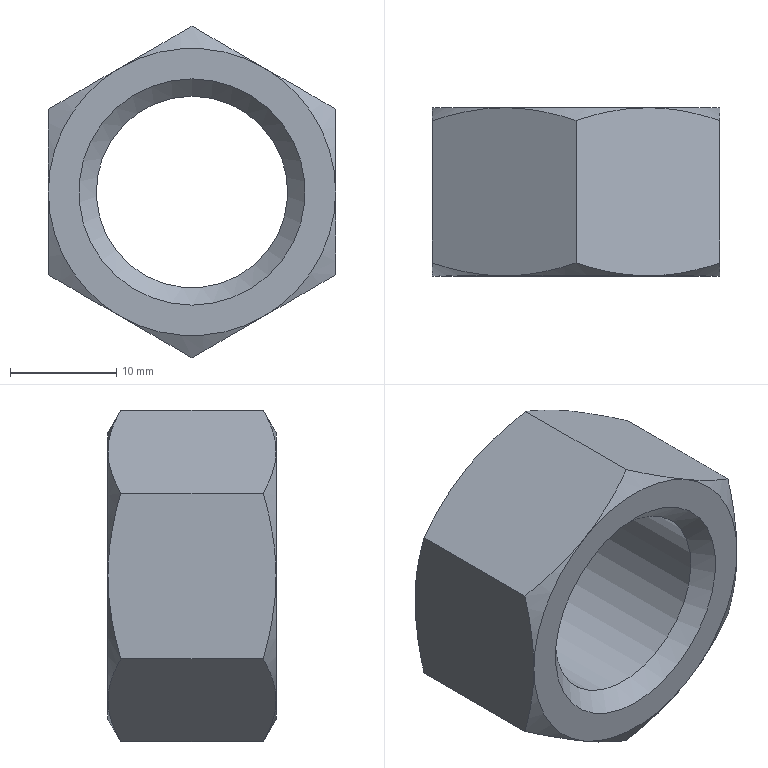Component | NX | GB-T6170_F-2000_M18X2_5 | 1 solid | 23 faces | volume 5751 mm3 | cone 14 | plane 8 | cylinder 1 | commonest cylinder face diameters 18 x1